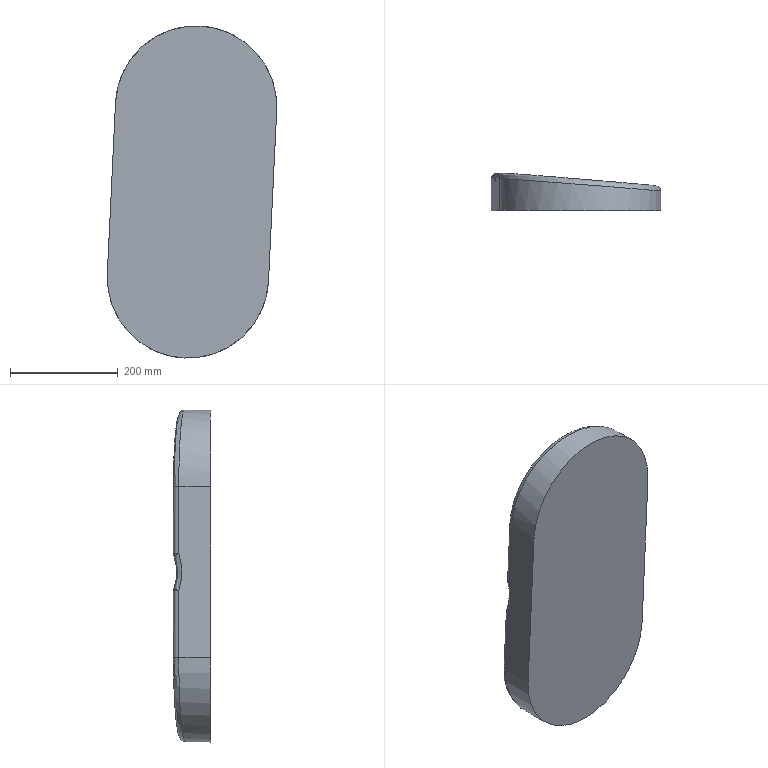Component | SolidWorks | 04-03BottomHousing-1 | 1 solid | 22 faces | box 315.25 x 69.13 x 617.63 mm | volume 9437459 mm3 | cylinder 9 | plane 5 | sphere 4 | spline 4 | commonest cylinder face diameters 20 x6 300 x2 180 x1
STEP:
#1=COLOUR_RGB('',0.7922,0.8196,0.9333);
#2=FILL_AREA_STYLE_COLOUR('',#1);
#3=FILL_AREA_STYLE('',(#2));
#4=SURFACE_STYLE_FILL_AREA(#3);
#5=SURFACE_SIDE_STYLE('',(#4));
#6=SURFACE_STYLE_USAGE(.BOTH.,#5);
#7=PRESENTATION_STYLE_ASSIGNMENT((#6));
#8=CARTESIAN_POINT('',(2.905,4.413,6.332));
#9=VERTEX_POINT('',#8);
#10=CARTESIAN_POINT('',(13.916,3.495,5.804));
#11=VERTEX_POINT('',#10);
#12=CARTESIAN_POINT('',(2.905,4.413,6.332));
#13=CARTESIAN_POINT('',(3.434,4.413,17.343));
#14=CARTESIAN_POINT('',(14.444,3.495,16.815));
#15=CARTESIAN_POINT('',(13.916,3.495,5.804));
#16=(BOUNDED_CURVE()B_SPLINE_CURVE(3,(#12,#13,#14,#15),.UNSPECIFIED.,.F.,.F.)B_SPLINE_CURVE_WITH_KNOTS((4,4),(3.142,6.283),.UNSPECIFIED.)CURVE()GEOMETRIC_REPRESENTATION_ITEM()RATIONAL_B_SPLINE_CURVE((1.,0.3333,0.3333,1.))REPRESENTATION_ITEM(''));
#17=EDGE_CURVE('',#9,#11,#16,.T.);
#18=ORIENTED_EDGE('',*,*,#17,.T.);
#19=CARTESIAN_POINT('',(13.68,3.495,0.8927));
#20=VERTEX_POINT('',#19);
#21=CARTESIAN_POINT('',(14.199,3.495,11.702));
#22=DIRECTION('',(-0.04795,-0.,-0.9988));
#23=VECTOR('',#22,39.37);
#24=LINE('',#21,#23);
#25=EDGE_CURVE('',#11,#20,#24,.T.);
#26=ORIENTED_EDGE('',*,*,#25,.T.);
#27=CARTESIAN_POINT('',(2.669,4.413,1.421));
#28=VERTEX_POINT('',#27);
#29=CARTESIAN_POINT('',(2.243,4.449,1.442));
#30=DIRECTION('',(-0.9954,0.08305,0.04778));
#31=VECTOR('',#30,39.37);
#32=LINE('',#29,#31);
#33=EDGE_CURVE('',#20,#28,#32,.T.);
#34=ORIENTED_EDGE('',*,*,#33,.T.);
#35=CARTESIAN_POINT('',(3.188,4.413,12.231));
#36=DIRECTION('',(0.04795,0.,0.9988));
#37=VECTOR('',#36,39.37);
#38=LINE('',#35,#37);
#39=EDGE_CURVE('',#28,#9,#38,.T.);
#40=ORIENTED_EDGE('',*,*,#39,.T.);
#41=EDGE_LOOP('',(#18,#26,#34,#40));
#42=FACE_OUTER_BOUND('',#41,.T.);
#43=CARTESIAN_POINT('',(2.762,4.449,12.251));
#44=DIRECTION('',(-0.08295,-0.9965,0.003982));
#45=DIRECTION('',(-0.9954,0.08305,0.04778));
#46=AXIS2_PLACEMENT_3D('',#43,#44,#45);
#47=PLANE('',#46);
#48=ADVANCED_FACE('',(#42),#47,.F.);
#49=CARTESIAN_POINT('',(13.316,3.495,-6.702));
#50=VERTEX_POINT('',#49);
#51=CARTESIAN_POINT('',(2.305,4.413,-6.173));
#52=VERTEX_POINT('',#51);
#53=CARTESIAN_POINT('',(13.316,3.495,-6.702));
#54=CARTESIAN_POINT('',(12.787,3.495,-17.713));
#55=CARTESIAN_POINT('',(1.776,4.413,-17.184));
#56=CARTESIAN_POINT('',(2.305,4.413,-6.173));
#57=(BOUNDED_CURVE()B_SPLINE_CURVE(3,(#53,#54,#55,#56),.UNSPECIFIED.,.F.,.F.)B_SPLINE_CURVE_WITH_KNOTS((4,4),(0.,3.142),.UNSPECIFIED.)CURVE()GEOMETRIC_REPRESENTATION_ITEM()RATIONAL_B_SPLINE_CURVE((1.,0.3333,0.3333,1.))REPRESENTATION_ITEM(''));
#58=EDGE_CURVE('',#50,#52,#57,.T.);
#59=ORIENTED_EDGE('',*,*,#58,.T.);
#60=CARTESIAN_POINT('',(2.54,4.413,-1.262));
#61=VERTEX_POINT('',#60);
#62=CARTESIAN_POINT('',(3.188,4.413,12.231));
#63=DIRECTION('',(0.04795,0.,0.9988));
#64=VECTOR('',#63,39.37);
#65=LINE('',#62,#64);
#66=EDGE_CURVE('',#52,#61,#65,.T.);
#67=ORIENTED_EDGE('',*,*,#66,.T.);
#68=CARTESIAN_POINT('',(13.551,3.495,-1.791));
#69=VERTEX_POINT('',#68);
#70=CARTESIAN_POINT('',(13.912,3.465,-1.808));
#71=DIRECTION('',(0.9954,-0.08305,-0.04778));
#72=VECTOR('',#71,39.37);
#73=LINE('',#70,#72);
#74=EDGE_CURVE('',#61,#69,#73,.T.);
#75=ORIENTED_EDGE('',*,*,#74,.T.);
#76=CARTESIAN_POINT('',(14.199,3.495,11.702));
#77=DIRECTION('',(-0.04795,-0.,-0.9988));
#78=VECTOR('',#77,39.37);
#79=LINE('',#76,#78);
#80=EDGE_CURVE('',#69,#50,#79,.T.);
#81=ORIENTED_EDGE('',*,*,#80,.T.);
#82=EDGE_LOOP('',(#59,#67,#75,#81));
#83=FACE_OUTER_BOUND('',#82,.T.);
#84=CARTESIAN_POINT('',(2.762,4.449,12.251));
#85=DIRECTION('',(-0.08295,-0.9965,0.003982));
#86=DIRECTION('',(-0.9954,0.08305,0.04778));
#87=AXIS2_PLACEMENT_3D('',#84,#85,#86);
#88=PLANE('',#87);
#89=ADVANCED_FACE('',(#83),#88,.F.);
#90=CARTESIAN_POINT('',(1.879,4.021,-6.153));
#91=VERTEX_POINT('',#90);
#92=CARTESIAN_POINT('',(1.879,1.693,-6.153));
#93=VERTEX_POINT('',#92);
#94=CARTESIAN_POINT('',(1.879,5.236,-6.153));
#95=DIRECTION('',(0.,-1.,0.));
#96=VECTOR('',#95,39.37);
#97=LINE('',#94,#96);
#98=EDGE_CURVE('',#91,#93,#97,.T.);
#99=ORIENTED_EDGE('',*,*,#98,.F.);
#100=CARTESIAN_POINT('',(13.676,3.102,-6.719));
#101=VERTEX_POINT('',#100);
#102=CARTESIAN_POINT('',(1.879,4.021,-6.153));
#103=CARTESIAN_POINT('',(1.312,4.021,-17.95));
#104=CARTESIAN_POINT('',(13.11,3.102,-18.516));
#105=CARTESIAN_POINT('',(13.676,3.102,-6.719));
#106=(BOUNDED_CURVE()B_SPLINE_CURVE(3,(#102,#103,#104,#105),.UNSPECIFIED.,.F.,.T.)B_SPLINE_CURVE_WITH_KNOTS((4,4),(3.142,6.283),.UNSPECIFIED.)CURVE()GEOMETRIC_REPRESENTATION_ITEM()RATIONAL_B_SPLINE_CURVE((1.,0.3333,0.3333,1.))REPRESENTATION_ITEM(''));
#107=EDGE_CURVE('',#91,#101,#106,.T.);
#108=ORIENTED_EDGE('',*,*,#107,.T.);
#109=CARTESIAN_POINT('',(13.676,1.693,-6.719));
#110=VERTEX_POINT('',#109);
#111=CARTESIAN_POINT('',(13.676,5.236,-6.719));
#112=DIRECTION('',(0.,-1.,0.));
#113=VECTOR('',#112,39.37);
#114=LINE('',#111,#113);
#115=EDGE_CURVE('',#101,#110,#114,.T.);
#116=ORIENTED_EDGE('',*,*,#115,.T.);
#117=CARTESIAN_POINT('',(7.777,1.693,-6.436));
#118=DIRECTION('',(-0.,1.,-0.));
#119=DIRECTION('',(0.9988,0.,-0.04795));
#120=AXIS2_PLACEMENT_3D('',#117,#118,#119);
#121=CIRCLE('',#120,5.906);
#122=EDGE_CURVE('',#110,#93,#121,.T.);
#123=ORIENTED_EDGE('',*,*,#122,.T.);
#124=EDGE_LOOP('',(#99,#108,#116,#123));
#125=FACE_OUTER_BOUND('',#124,.T.);
#126=CARTESIAN_POINT('',(7.777,5.236,-6.436));
#127=DIRECTION('',(0.,-1.,0.));
#128=DIRECTION('',(-0.9988,-0.,0.04795));
#129=AXIS2_PLACEMENT_3D('',#126,#127,#128);
#130=CYLINDRICAL_SURFACE('',#129,5.906);
#131=ADVANCED_FACE('',(#125),#130,.T.);
#132=CARTESIAN_POINT('',(2.479,4.021,6.353));
#133=VERTEX_POINT('',#132);
#134=CARTESIAN_POINT('',(2.479,1.693,6.353));
#135=VERTEX_POINT('',#134);
#136=CARTESIAN_POINT('',(2.479,5.236,6.353));
#137=DIRECTION('',(0.,-1.,0.));
#138=VECTOR('',#137,39.37);
#139=LINE('',#136,#138);
#140=EDGE_CURVE('',#133,#135,#139,.T.);
#141=ORIENTED_EDGE('',*,*,#140,.F.);
#142=CARTESIAN_POINT('',(2.243,4.021,1.442));
#143=VERTEX_POINT('',#142);
#144=CARTESIAN_POINT('',(1.879,4.021,-6.153));
#145=DIRECTION('',(-0.04795,-0.,-0.9988));
#146=VECTOR('',#145,39.37);
#147=LINE('',#144,#146);
#148=EDGE_CURVE('',#133,#143,#147,.T.);
#149=ORIENTED_EDGE('',*,*,#148,.T.);
#150=CARTESIAN_POINT('',(2.114,4.021,-1.242));
#151=VERTEX_POINT('',#150);
#152=CARTESIAN_POINT('',(2.243,4.021,1.442));
#153=CARTESIAN_POINT('',(2.201,3.702,0.5659));
#154=CARTESIAN_POINT('',(2.157,3.702,-0.3658));
#155=CARTESIAN_POINT('',(2.114,4.021,-1.242));
#156=(BOUNDED_CURVE()B_SPLINE_CURVE(3,(#152,#153,#154,#155),.UNSPECIFIED.,.F.,.F.)B_SPLINE_CURVE_WITH_KNOTS((4,4),(2.793,3.49),.UNSPECIFIED.)CURVE()GEOMETRIC_REPRESENTATION_ITEM()RATIONAL_B_SPLINE_CURVE((1.,0.96,0.96,1.))REPRESENTATION_ITEM(''));
#157=EDGE_CURVE('',#143,#151,#156,.T.);
#158=ORIENTED_EDGE('',*,*,#157,.T.);
#159=CARTESIAN_POINT('',(1.879,4.021,-6.153));
#160=DIRECTION('',(-0.04795,-0.,-0.9988));
#161=VECTOR('',#160,39.37);
#162=LINE('',#159,#161);
#163=EDGE_CURVE('',#151,#91,#162,.T.);
#164=ORIENTED_EDGE('',*,*,#163,.T.);
#165=ORIENTED_EDGE('',*,*,#98,.T.);
#166=CARTESIAN_POINT('',(1.879,1.693,-6.153));
#167=DIRECTION('',(0.04795,0.,0.9988));
#168=VECTOR('',#167,39.37);
#169=LINE('',#166,#168);
#170=EDGE_CURVE('',#93,#135,#169,.T.);
#171=ORIENTED_EDGE('',*,*,#170,.T.);
#172=EDGE_LOOP('',(#141,#149,#158,#164,#165,#171));
#173=FACE_OUTER_BOUND('',#172,.T.);
#174=CARTESIAN_POINT('',(1.879,5.236,-6.153));
#175=DIRECTION('',(0.9988,0.,-0.04795));
#176=DIRECTION('',(-0.04795,-0.,-0.9988));
#177=AXIS2_PLACEMENT_3D('',#174,#175,#176);
#178=PLANE('',#177);
#179=ADVANCED_FACE('',(#173),#178,.F.);
#180=CARTESIAN_POINT('',(14.276,3.102,5.786));
#181=VERTEX_POINT('',#180);
#182=CARTESIAN_POINT('',(14.276,1.693,5.786));
#183=VERTEX_POINT('',#182);
#184=CARTESIAN_POINT('',(14.276,5.236,5.786));
#185=DIRECTION('',(0.,-1.,0.));
#186=VECTOR('',#185,39.37);
#187=LINE('',#184,#186);
#188=EDGE_CURVE('',#181,#183,#187,.T.);
#189=ORIENTED_EDGE('',*,*,#188,.F.);
#190=CARTESIAN_POINT('',(14.276,3.102,5.786));
#191=CARTESIAN_POINT('',(14.843,3.102,17.584));
#192=CARTESIAN_POINT('',(3.045,4.021,18.15));
#193=CARTESIAN_POINT('',(2.479,4.021,6.353));
#194=(BOUNDED_CURVE()B_SPLINE_CURVE(3,(#190,#191,#192,#193),.UNSPECIFIED.,.F.,.F.)B_SPLINE_CURVE_WITH_KNOTS((4,4),(0.,3.142),.UNSPECIFIED.)CURVE()GEOMETRIC_REPRESENTATION_ITEM()RATIONAL_B_SPLINE_CURVE((1.,0.3333,0.3333,1.))REPRESENTATION_ITEM(''));
#195=EDGE_CURVE('',#181,#133,#194,.T.);
#196=ORIENTED_EDGE('',*,*,#195,.T.);
#197=ORIENTED_EDGE('',*,*,#140,.T.);
#198=CARTESIAN_POINT('',(8.378,1.693,6.07));
#199=DIRECTION('',(-0.,1.,-0.));
#200=DIRECTION('',(0.9988,0.,-0.04795));
#201=AXIS2_PLACEMENT_3D('',#198,#199,#200);
#202=CIRCLE('',#201,5.906);
#203=EDGE_CURVE('',#135,#183,#202,.T.);
#204=ORIENTED_EDGE('',*,*,#203,.T.);
#205=EDGE_LOOP('',(#189,#196,#197,#204));
#206=FACE_OUTER_BOUND('',#205,.T.);
#207=CARTESIAN_POINT('',(8.378,5.236,6.07));
#208=DIRECTION('',(0.,-1.,0.));
#209=DIRECTION('',(-0.9988,-0.,0.04795));
#210=AXIS2_PLACEMENT_3D('',#207,#208,#209);
#211=CYLINDRICAL_SURFACE('',#210,5.906);
#212=ADVANCED_FACE('',(#206),#211,.T.);
#213=CARTESIAN_POINT('',(13.912,3.102,-1.808));
#214=VERTEX_POINT('',#213);
#215=CARTESIAN_POINT('',(14.041,3.102,0.8754));
#216=VERTEX_POINT('',#215);
#217=CARTESIAN_POINT('',(13.912,3.102,-1.808));
#218=CARTESIAN_POINT('',(13.954,2.783,-0.9321));
#219=CARTESIAN_POINT('',(13.999,2.783,-0.0004051));
#220=CARTESIAN_POINT('',(14.041,3.102,0.8754));
#221=(BOUNDED_CURVE()B_SPLINE_CURVE(3,(#217,#218,#219,#220),.UNSPECIFIED.,.F.,.F.)B_SPLINE_CURVE_WITH_KNOTS((4,4),(2.793,3.49),.UNSPECIFIED.)CURVE()GEOMETRIC_REPRESENTATION_ITEM()RATIONAL_B_SPLINE_CURVE((1.,0.96,0.96,1.))REPRESENTATION_ITEM(''));
#222=EDGE_CURVE('',#214,#216,#221,.T.);
#223=ORIENTED_EDGE('',*,*,#222,.T.);
#224=CARTESIAN_POINT('',(13.676,3.102,-6.719));
#225=DIRECTION('',(0.04795,0.,0.9988));
#226=VECTOR('',#225,39.37);
#227=LINE('',#224,#226);
#228=EDGE_CURVE('',#216,#181,#227,.T.);
#229=ORIENTED_EDGE('',*,*,#228,.T.);
#230=ORIENTED_EDGE('',*,*,#188,.T.);
#231=CARTESIAN_POINT('',(13.676,1.693,-6.719));
#232=DIRECTION('',(-0.04795,-0.,-0.9988));
#233=VECTOR('',#232,39.37);
#234=LINE('',#231,#233);
#235=EDGE_CURVE('',#183,#110,#234,.T.);
#236=ORIENTED_EDGE('',*,*,#235,.T.);
#237=ORIENTED_EDGE('',*,*,#115,.F.);
#238=CARTESIAN_POINT('',(13.676,3.102,-6.719));
#239=DIRECTION('',(0.04795,0.,0.9988));
#240=VECTOR('',#239,39.37);
#241=LINE('',#238,#240);
#242=EDGE_CURVE('',#101,#214,#241,.T.);
#243=ORIENTED_EDGE('',*,*,#242,.T.);
#244=EDGE_LOOP('',(#223,#229,#230,#236,#237,#243));
#245=FACE_OUTER_BOUND('',#244,.T.);
#246=CARTESIAN_POINT('',(13.676,5.236,-6.719));
#247=DIRECTION('',(-0.9988,-0.,0.04795));
#248=DIRECTION('',(0.04795,0.,0.9988));
#249=AXIS2_PLACEMENT_3D('',#246,#247,#248);
#250=PLANE('',#249);
#251=ADVANCED_FACE('',(#245),#250,.F.);
#252=ORIENTED_EDGE('',*,*,#122,.F.);
#253=ORIENTED_EDGE('',*,*,#235,.F.);
#254=ORIENTED_EDGE('',*,*,#203,.F.);
#255=ORIENTED_EDGE('',*,*,#170,.F.);
#256=EDGE_LOOP('',(#252,#253,#254,#255));
#257=FACE_OUTER_BOUND('',#256,.T.);
#258=CARTESIAN_POINT('',(7.777,1.693,-6.436));
#259=DIRECTION('',(-0.,1.,-0.));
#260=DIRECTION('',(0.9988,0.,-0.04795));
#261=AXIS2_PLACEMENT_3D('',#258,#259,#260);
#262=PLANE('',#261);
#263=ADVANCED_FACE('',(#257),#262,.F.);
#264=CARTESIAN_POINT('',(2.545,4.39,-1.128));
#265=VERTEX_POINT('',#264);
#266=CARTESIAN_POINT('',(2.661,4.39,1.287));
#267=VERTEX_POINT('',#266);
#268=CARTESIAN_POINT('',(2.545,4.39,-1.128));
#269=CARTESIAN_POINT('',(2.585,4.102,-0.3397));
#270=CARTESIAN_POINT('',(2.626,4.102,0.4989));
#271=CARTESIAN_POINT('',(2.661,4.39,1.287));
#272=(BOUNDED_CURVE()B_SPLINE_CURVE(3,(#268,#269,#270,#271),.UNSPECIFIED.,.F.,.T.)B_SPLINE_CURVE_WITH_KNOTS((4,4),(2.793,3.49),.UNSPECIFIED.)CURVE()GEOMETRIC_REPRESENTATION_ITEM()RATIONAL_B_SPLINE_CURVE((1.,0.96,0.96,1.))REPRESENTATION_ITEM(''));
#273=EDGE_CURVE('',#265,#267,#272,.T.);
#274=ORIENTED_EDGE('',*,*,#273,.T.);
#275=CARTESIAN_POINT('',(13.672,3.471,0.7586));
#276=VERTEX_POINT('',#275);
#277=CARTESIAN_POINT('',(1.297,4.504,1.353));
#278=DIRECTION('',(0.9954,-0.08305,-0.04778));
#279=VECTOR('',#278,39.37);
#280=LINE('',#277,#279);
#281=EDGE_CURVE('',#267,#276,#280,.T.);
#282=ORIENTED_EDGE('',*,*,#281,.T.);
#283=CARTESIAN_POINT('',(13.556,3.471,-1.656));
#284=VERTEX_POINT('',#283);
#285=CARTESIAN_POINT('',(13.672,3.471,0.7586));
#286=CARTESIAN_POINT('',(13.637,3.183,-0.02971));
#287=CARTESIAN_POINT('',(13.596,3.183,-0.8683));
#288=CARTESIAN_POINT('',(13.556,3.471,-1.656));
#289=(BOUNDED_CURVE()B_SPLINE_CURVE(3,(#285,#286,#287,#288),.UNSPECIFIED.,.F.,.F.)B_SPLINE_CURVE_WITH_KNOTS((4,4),(2.793,3.49),.UNSPECIFIED.)CURVE()GEOMETRIC_REPRESENTATION_ITEM()RATIONAL_B_SPLINE_CURVE((1.,0.96,0.96,1.))REPRESENTATION_ITEM(''));
#290=EDGE_CURVE('',#276,#284,#289,.T.);
#291=ORIENTED_EDGE('',*,*,#290,.T.);
#292=CARTESIAN_POINT('',(1.181,4.504,-1.062));
#293=DIRECTION('',(-0.9954,0.08305,0.04778));
#294=VECTOR('',#293,39.37);
#295=LINE('',#292,#294);
#296=EDGE_CURVE('',#284,#265,#295,.T.);
#297=ORIENTED_EDGE('',*,*,#296,.T.);
#298=EDGE_LOOP('',(#274,#282,#291,#297));
#299=FACE_OUTER_BOUND('',#298,.T.);
#300=CARTESIAN_POINT('',(1.515,7.823,0.1319));
#301=DIRECTION('',(-0.9954,0.08305,0.04778));
#302=DIRECTION('',(0.08295,0.9965,-0.003982));
#303=AXIS2_PLACEMENT_3D('',#300,#301,#302);
#304=CYLINDRICAL_SURFACE('',#303,3.543);
#305=ADVANCED_FACE('',(#299),#304,.F.);
#306=CARTESIAN_POINT('',(2.508,4.021,-1.26));
#307=DIRECTION('',(0.04795,-0.,0.9988));
#308=DIRECTION('',(0.9988,0.,-0.04795));
#309=AXIS2_PLACEMENT_3D('',#306,#307,#308);
#310=CIRCLE('',#309,0.3937);
#311=EDGE_CURVE('',#61,#151,#310,.T.);
#312=ORIENTED_EDGE('',*,*,#311,.F.);
#313=ORIENTED_EDGE('',*,*,#66,.F.);
#314=CARTESIAN_POINT('',(2.272,4.021,-6.171));
#315=DIRECTION('',(-0.04795,-0.,-0.9988));
#316=DIRECTION('',(-0.9988,0.,0.04795));
#317=AXIS2_PLACEMENT_3D('',#314,#315,#316);
#318=CIRCLE('',#317,0.3937);
#319=EDGE_CURVE('',#91,#52,#318,.T.);
#320=ORIENTED_EDGE('',*,*,#319,.F.);
#321=ORIENTED_EDGE('',*,*,#163,.F.);
#322=EDGE_LOOP('',(#312,#313,#320,#321));
#323=FACE_OUTER_BOUND('',#322,.T.);
#324=CARTESIAN_POINT('',(2.272,4.021,-6.171));
#325=DIRECTION('',(-0.04795,-0.,-0.9988));
#326=DIRECTION('',(-0.9988,0.,0.04795));
#327=AXIS2_PLACEMENT_3D('',#324,#325,#326);
#328=CYLINDRICAL_SURFACE('',#327,0.3937);
#329=ADVANCED_FACE('',(#323),#328,.T.);
#330=CARTESIAN_POINT('',(2.508,4.021,-1.26));
#331=DIRECTION('',(0.9954,-0.08305,-0.04778));
#332=DIRECTION('',(0.08295,0.9965,-0.003982));
#333=AXIS2_PLACEMENT_3D('',#330,#331,#332);
#334=CIRCLE('',#333,0.3937);
#335=EDGE_CURVE('',#61,#265,#334,.T.);
#336=ORIENTED_EDGE('',*,*,#335,.F.);
#337=ORIENTED_EDGE('',*,*,#311,.T.);
#338=CARTESIAN_POINT('',(2.508,4.021,-1.26));
#339=DIRECTION('',(0.04505,-0.3422,0.9385));
#340=DIRECTION('',(0.01641,0.9396,0.3418));
#341=AXIS2_PLACEMENT_3D('',#338,#339,#340);
#342=CIRCLE('',#341,0.3937);
#343=EDGE_CURVE('',#265,#151,#342,.T.);
#344=ORIENTED_EDGE('',*,*,#343,.F.);
#345=EDGE_LOOP('',(#336,#337,#344));
#346=FACE_OUTER_BOUND('',#345,.T.);
#347=CARTESIAN_POINT('',(2.508,4.021,-1.26));
#348=DIRECTION('',(-0.,1.,0.));
#349=DIRECTION('',(-0.04795,0.,-0.9988));
#350=AXIS2_PLACEMENT_3D('',#347,#348,#349);
#351=SPHERICAL_SURFACE('',#350,0.3937);
#352=ADVANCED_FACE('',(#346),#351,.T.);
#353=ORIENTED_EDGE('',*,*,#319,.T.);
#354=ORIENTED_EDGE('',*,*,#58,.F.);
#355=CARTESIAN_POINT('',(13.283,3.102,-6.7));
#356=DIRECTION('',(0.04795,0.,0.9988));
#357=DIRECTION('',(0.9988,0.,-0.04795));
#358=AXIS2_PLACEMENT_3D('',#355,#356,#357);
#359=CIRCLE('',#358,0.3937);
#360=EDGE_CURVE('',#101,#50,#359,.T.);
#361=ORIENTED_EDGE('',*,*,#360,.F.);
#362=ORIENTED_EDGE('',*,*,#107,.F.);
#363=EDGE_LOOP('',(#353,#354,#361,#362));
#364=FACE_OUTER_BOUND('',#363,.T.);
#365=CARTESIAN_POINT('',(2.305,4.413,-6.173));
#366=CARTESIAN_POINT('',(1.879,4.449,-6.153));
#367=CARTESIAN_POINT('',(1.879,4.021,-6.153));
#368=CARTESIAN_POINT('',(2.287,4.413,-6.533));
#369=CARTESIAN_POINT('',(1.86,4.449,-6.541));
#370=CARTESIAN_POINT('',(1.86,4.021,-6.539));
#371=CARTESIAN_POINT('',(2.306,4.41,-6.895));
#372=CARTESIAN_POINT('',(1.88,4.446,-6.931));
#373=CARTESIAN_POINT('',(1.88,4.018,-6.927));
#374=CARTESIAN_POINT('',(2.412,4.399,-7.609));
#375=CARTESIAN_POINT('',(1.996,4.433,-7.7));
#376=CARTESIAN_POINT('',(1.994,4.006,-7.691));
#377=CARTESIAN_POINT('',(2.501,4.39,-7.96));
#378=CARTESIAN_POINT('',(2.092,4.423,-8.078));
#379=CARTESIAN_POINT('',(2.089,3.997,-8.068));
#380=CARTESIAN_POINT('',(2.744,4.367,-8.64));
#381=CARTESIAN_POINT('',(2.356,4.398,-8.809));
#382=CARTESIAN_POINT('',(2.35,3.974,-8.795));
#383=CARTESIAN_POINT('',(2.9,4.353,-8.967));
#384=CARTESIAN_POINT('',(2.524,4.383,-9.161));
#385=CARTESIAN_POINT('',(2.516,3.96,-9.146));
#386=CARTESIAN_POINT('',(3.271,4.319,-9.585));
#387=CARTESIAN_POINT('',(2.926,4.347,-9.826));
#388=CARTESIAN_POINT('',(2.915,3.927,-9.809));
#389=CARTESIAN_POINT('',(3.488,4.3,-9.876));
#390=CARTESIAN_POINT('',(3.16,4.326,-10.138));
#391=CARTESIAN_POINT('',(3.146,3.908,-10.12));
#392=CARTESIAN_POINT('',(3.973,4.257,-10.41));
#393=CARTESIAN_POINT('',(3.684,4.28,-10.71));
#394=CARTESIAN_POINT('',(3.666,3.865,-10.693));
#395=CARTESIAN_POINT('',(4.242,4.234,-10.654));
#396=CARTESIAN_POINT('',(3.974,4.255,-10.97));
#397=CARTESIAN_POINT('',(3.954,3.842,-10.953));
#398=CARTESIAN_POINT('',(4.822,4.184,-11.083));
#399=CARTESIAN_POINT('',(4.6,4.201,-11.428));
#400=CARTESIAN_POINT('',(4.576,3.792,-11.413));
#401=CARTESIAN_POINT('',(5.133,4.158,-11.269));
#402=CARTESIAN_POINT('',(4.935,4.173,-11.627));
#403=CARTESIAN_POINT('',(4.909,3.765,-11.612));
#404=CARTESIAN_POINT('',(5.785,4.102,-11.576));
#405=CARTESIAN_POINT('',(5.637,4.113,-11.953));
#406=CARTESIAN_POINT('',(5.608,3.71,-11.942));
#407=CARTESIAN_POINT('',(6.127,4.073,-11.698));
#408=CARTESIAN_POINT('',(6.004,4.082,-12.082));
#409=CARTESIAN_POINT('',(5.974,3.681,-12.072));
#410=CARTESIAN_POINT('',(6.827,4.014,-11.873));
#411=CARTESIAN_POINT('',(6.755,4.018,-12.265));
#412=CARTESIAN_POINT('',(6.724,3.622,-12.259));
#413=CARTESIAN_POINT('',(7.185,3.984,-11.925));
#414=CARTESIAN_POINT('',(7.14,3.986,-12.32));
#415=CARTESIAN_POINT('',(7.108,3.592,-12.316));
#416=CARTESIAN_POINT('',(7.906,3.924,-11.96));
#417=CARTESIAN_POINT('',(7.912,3.922,-12.352));
#418=CARTESIAN_POINT('',(7.88,3.532,-12.353));
#419=CARTESIAN_POINT('',(8.268,3.894,-11.942));
#420=CARTESIAN_POINT('',(8.299,3.89,-12.331));
#421=CARTESIAN_POINT('',(8.268,3.502,-12.333));
#422=CARTESIAN_POINT('',(8.982,3.835,-11.835));
#423=CARTESIAN_POINT('',(9.062,3.827,-12.213));
#424=CARTESIAN_POINT('',(9.033,3.443,-12.219));
#425=CARTESIAN_POINT('',(9.333,3.806,-11.747));
#426=CARTESIAN_POINT('',(9.438,3.796,-12.116));
#427=CARTESIAN_POINT('',(9.409,3.414,-12.124));
#428=CARTESIAN_POINT('',(10.012,3.75,-11.503));
#429=CARTESIAN_POINT('',(10.162,3.737,-11.852));
#430=CARTESIAN_POINT('',(10.137,3.358,-11.863));
#431=CARTESIAN_POINT('',(10.34,3.724,-11.348));
#432=CARTESIAN_POINT('',(10.511,3.708,-11.685));
#433=CARTESIAN_POINT('',(10.488,3.331,-11.697));
#434=CARTESIAN_POINT('',(10.958,3.674,-10.976));
#435=CARTESIAN_POINT('',(11.17,3.655,-11.285));
#436=CARTESIAN_POINT('',(11.15,3.281,-11.299));
#437=CARTESIAN_POINT('',(11.249,3.65,-10.76));
#438=CARTESIAN_POINT('',(11.48,3.63,-11.053));
#439=CARTESIAN_POINT('',(11.462,3.258,-11.067));
#440=CARTESIAN_POINT('',(11.783,3.608,-10.275));
#441=CARTESIAN_POINT('',(12.048,3.585,-10.533));
#442=CARTESIAN_POINT('',(12.034,3.216,-10.547));
#443=CARTESIAN_POINT('',(12.026,3.589,-10.006));
#444=CARTESIAN_POINT('',(12.307,3.564,-10.245));
#445=CARTESIAN_POINT('',(12.295,3.196,-10.259));
#446=CARTESIAN_POINT('',(12.455,3.555,-9.426));
#447=CARTESIAN_POINT('',(12.763,3.529,-9.625));
#448=CARTESIAN_POINT('',(12.755,3.163,-9.638));
#449=CARTESIAN_POINT('',(12.641,3.541,-9.115));
#450=CARTESIAN_POINT('',(12.96,3.514,-9.293));
#451=CARTESIAN_POINT('',(12.954,3.149,-9.304));
#452=CARTESIAN_POINT('',(12.949,3.518,-8.462));
#453=CARTESIAN_POINT('',(13.287,3.489,-8.596));
#454=CARTESIAN_POINT('',(13.284,3.126,-8.605));
#455=CARTESIAN_POINT('',(13.071,3.509,-8.121));
#456=CARTESIAN_POINT('',(13.416,3.48,-8.232));
#457=CARTESIAN_POINT('',(13.414,3.117,-8.239));
#458=CARTESIAN_POINT('',(13.246,3.498,-7.421));
#459=CARTESIAN_POINT('',(13.602,3.468,-7.485));
#460=CARTESIAN_POINT('',(13.601,3.105,-7.489));
#461=CARTESIAN_POINT('',(13.298,3.495,-7.062));
#462=CARTESIAN_POINT('',(13.658,3.465,-7.103));
#463=CARTESIAN_POINT('',(13.658,3.102,-7.105));
#464=CARTESIAN_POINT('',(13.316,3.495,-6.702));
#465=CARTESIAN_POINT('',(13.676,3.465,-6.719));
#466=CARTESIAN_POINT('',(13.676,3.102,-6.719));
#467=(BOUNDED_SURFACE()B_SPLINE_SURFACE(3,2,((#365,#366,#367),(#368,#369,#370),(#371,#372,#373),(#374,#375,#376),(#377,#378,#379),(#380,#381,#382),(#383,#384,#385),(#386,#387,#388),(#389,#390,#391),(#392,#393,#394),(#395,#396,#397),(#398,#399,#400),(#401,#402,#403),(#404,#405,#406),(#407,#408,#409),(#410,#411,#412),(#413,#414,#415),(#416,#417,#418),(#419,#420,#421),(#422,#423,#424),(#425,#426,#427),(#428,#429,#430),(#431,#432,#433),(#434,#435,#436),(#437,#438,#439),(#440,#441,#442),(#443,#444,#445),(#446,#447,#448),(#449,#450,#451),(#452,#453,#454),(#455,#456,#457),(#458,#459,#460),(#461,#462,#463),(#464,#465,#466)),.UNSPECIFIED.,.F.,.F.,.T.)B_SPLINE_SURFACE_WITH_KNOTS((4,2,2,2,2,2,2,2,2,2,2,2,2,2,2,2,4),(3,3),(3.142,3.338,3.534,3.731,3.927,4.123,4.32,4.516,4.712,4.909,5.105,5.301,5.498,5.694,5.89,6.087,6.283),(0.,1.),.UNSPECIFIED.)GEOMETRIC_REPRESENTATION_ITEM()RATIONAL_B_SPLINE_SURFACE(((1.,0.6771,1.),(1.,0.6771,1.),(1.,0.6773,1.),(1.,0.6781,1.),(1.,0.6787,1.),(1.,0.6802,1.),(1.,0.6812,1.),(1.,0.6834,1.),(1.,0.6846,1.),(1.,0.6874,1.),(1.,0.689,1.),(1.,0.6922,1.),(1.,0.694,1.),(1.,0.6976,1.),(1.,0.6995,1.),(1.,0.7033,1.),(1.,0.7052,1.),(1.,0.709,1.),(1.,0.7109,1.),(1.,0.7147,1.),(1.,0.7165,1.),(1.,0.72,1.),(1.,0.7217,1.),(1.,0.7248,1.),(1.,0.7263,1.),(1.,0.7289,1.),(1.,0.7301,1.),(1.,0.7321,1.),(1.,0.733,1.),(1.,0.7344,1.),(1.,0.735,1.),(1.,0.7357,1.),(1.,0.7359,1.),(1.,0.7359,1.)))REPRESENTATION_ITEM('')SURFACE());
#468=ADVANCED_FACE('',(#364),#467,.T.);
#469=ORIENTED_EDGE('',*,*,#343,.T.);
#470=ORIENTED_EDGE('',*,*,#157,.F.);
#471=CARTESIAN_POINT('',(2.637,4.021,1.423));
#472=DIRECTION('',(0.04505,0.3422,0.9385));
#473=DIRECTION('',(0.01641,-0.9396,0.3418));
#474=AXIS2_PLACEMENT_3D('',#471,#472,#473);
#475=CIRCLE('',#474,0.3937);
#476=EDGE_CURVE('',#267,#143,#475,.T.);
#477=ORIENTED_EDGE('',*,*,#476,.F.);
#478=ORIENTED_EDGE('',*,*,#273,.F.);
#479=EDGE_LOOP('',(#469,#470,#477,#478));
#480=FACE_OUTER_BOUND('',#479,.T.);
#481=CARTESIAN_POINT('',(2.661,4.39,1.287));
#482=CARTESIAN_POINT('',(2.236,4.421,1.296));
#483=CARTESIAN_POINT('',(2.243,4.021,1.442));
#484=CARTESIAN_POINT('',(2.652,4.319,1.094));
#485=CARTESIAN_POINT('',(2.227,4.352,1.105));
#486=CARTESIAN_POINT('',(2.233,3.943,1.227));
#487=CARTESIAN_POINT('',(2.643,4.266,0.895));
#488=CARTESIAN_POINT('',(2.218,4.299,0.9073));
#489=CARTESIAN_POINT('',(2.222,3.883,1.006));
#490=CARTESIAN_POINT('',(2.624,4.194,0.4904));
#491=CARTESIAN_POINT('',(2.198,4.229,0.5066));
#492=CARTESIAN_POINT('',(2.201,3.804,0.5565));
#493=CARTESIAN_POINT('',(2.615,4.176,0.285));
#494=CARTESIAN_POINT('',(2.189,4.212,0.3034));
#495=CARTESIAN_POINT('',(2.19,3.784,0.3283));
#496=CARTESIAN_POINT('',(2.595,4.176,-0.1257));
#497=CARTESIAN_POINT('',(2.169,4.212,-0.1032));
#498=CARTESIAN_POINT('',(2.168,3.784,-0.1281));
#499=CARTESIAN_POINT('',(2.585,4.194,-0.3311));
#500=CARTESIAN_POINT('',(2.159,4.229,-0.3064));
#501=CARTESIAN_POINT('',(2.157,3.804,-0.3563));
#502=CARTESIAN_POINT('',(2.565,4.266,-0.7356));
#503=CARTESIAN_POINT('',(2.14,4.299,-0.7071));
#504=CARTESIAN_POINT('',(2.135,3.883,-0.8058));
#505=CARTESIAN_POINT('',(2.555,4.319,-0.9347));
#506=CARTESIAN_POINT('',(2.131,4.352,-0.9044));
#507=CARTESIAN_POINT('',(2.125,3.943,-1.027));
#508=CARTESIAN_POINT('',(2.545,4.39,-1.128));
#509=CARTESIAN_POINT('',(2.121,4.421,-1.096));
#510=CARTESIAN_POINT('',(2.114,4.021,-1.242));
#511=(BOUNDED_SURFACE()B_SPLINE_SURFACE(3,2,((#481,#482,#483),(#484,#485,#486),(#487,#488,#489),(#490,#491,#492),(#493,#494,#495),(#496,#497,#498),(#499,#500,#501),(#502,#503,#504),(#505,#506,#507),(#508,#509,#510)),.UNSPECIFIED.,.F.,.F.,.T.)B_SPLINE_SURFACE_WITH_KNOTS((4,2,2,2,4),(3,3),(2.793,2.968,3.142,3.316,3.49),(0.,1.),.UNSPECIFIED.)GEOMETRIC_REPRESENTATION_ITEM()RATIONAL_B_SPLINE_SURFACE(((1.,0.6789,1.),(1.,0.6783,1.),(1.,0.6779,1.),(1.,0.6773,1.),(1.,0.6771,1.),(1.,0.6771,1.),(1.,0.6773,1.),(1.,0.6779,1.),(1.,0.6783,1.),(1.,0.6789,1.)))REPRESENTATION_ITEM('')SURFACE());
#512=ADVANCED_FACE('',(#480),#511,.T.);
#513=ORIENTED_EDGE('',*,*,#335,.T.);
#514=ORIENTED_EDGE('',*,*,#296,.F.);
#515=CARTESIAN_POINT('',(13.519,3.102,-1.789));
#516=DIRECTION('',(0.9954,-0.08305,-0.04778));
#517=DIRECTION('',(-0.08295,-0.9965,0.003982));
#518=AXIS2_PLACEMENT_3D('',#515,#516,#517);
#519=CIRCLE('',#518,0.3937);
#520=EDGE_CURVE('',#69,#284,#519,.T.);
#521=ORIENTED_EDGE('',*,*,#520,.F.);
#522=ORIENTED_EDGE('',*,*,#74,.F.);
#523=EDGE_LOOP('',(#513,#514,#521,#522));
#524=FACE_OUTER_BOUND('',#523,.T.);
#525=CARTESIAN_POINT('',(1.144,4.135,-1.195));
#526=DIRECTION('',(-0.9954,0.08305,0.04778));
#527=DIRECTION('',(0.08295,0.9965,-0.003982));
#528=AXIS2_PLACEMENT_3D('',#525,#526,#527);
#529=CYLINDRICAL_SURFACE('',#528,0.3937);
#530=ADVANCED_FACE('',(#524),#529,.T.);
#531=ORIENTED_EDGE('',*,*,#360,.T.);
#532=ORIENTED_EDGE('',*,*,#80,.F.);
#533=CARTESIAN_POINT('',(13.519,3.102,-1.789));
#534=DIRECTION('',(0.04795,0.,0.9988));
#535=DIRECTION('',(0.,-1.,0.));
#536=AXIS2_PLACEMENT_3D('',#533,#534,#535);
#537=CIRCLE('',#536,0.3937);
#538=EDGE_CURVE('',#214,#69,#537,.T.);
#539=ORIENTED_EDGE('',*,*,#538,.F.);
#540=ORIENTED_EDGE('',*,*,#242,.F.);
#541=EDGE_LOOP('',(#531,#532,#539,#540));
#542=FACE_OUTER_BOUND('',#541,.T.);
#543=CARTESIAN_POINT('',(14.166,3.102,11.704));
#544=DIRECTION('',(-0.04795,-0.,-0.9988));
#545=DIRECTION('',(-0.9988,0.,0.04795));
#546=AXIS2_PLACEMENT_3D('',#543,#544,#545);
#547=CYLINDRICAL_SURFACE('',#546,0.3937);
#548=ADVANCED_FACE('',(#542),#547,.T.);
#549=CARTESIAN_POINT('',(2.637,4.021,1.423));
#550=DIRECTION('',(0.9954,-0.08305,-0.04778));
#551=DIRECTION('',(0.08295,0.9965,-0.003982));
#552=AXIS2_PLACEMENT_3D('',#549,#550,#551);
#553=CIRCLE('',#552,0.3937);
#554=EDGE_CURVE('',#267,#28,#553,.T.);
#555=ORIENTED_EDGE('',*,*,#554,.F.);
#556=ORIENTED_EDGE('',*,*,#476,.T.);
#557=CARTESIAN_POINT('',(2.637,4.021,1.423));
#558=DIRECTION('',(0.04795,-0.,0.9988));
#559=DIRECTION('',(0.,1.,0.));
#560=AXIS2_PLACEMENT_3D('',#557,#558,#559);
#561=CIRCLE('',#560,0.3937);
#562=EDGE_CURVE('',#28,#143,#561,.T.);
#563=ORIENTED_EDGE('',*,*,#562,.F.);
#564=EDGE_LOOP('',(#555,#556,#563));
#565=FACE_OUTER_BOUND('',#564,.T.);
#566=CARTESIAN_POINT('',(2.637,4.021,1.423));
#567=DIRECTION('',(-0.,1.,0.));
#568=DIRECTION('',(-0.04795,0.,-0.9988));
#569=AXIS2_PLACEMENT_3D('',#566,#567,#568);
#570=SPHERICAL_SURFACE('',#569,0.3937);
#571=ADVANCED_FACE('',(#565),#570,.T.);
#572=ORIENTED_EDGE('',*,*,#538,.T.);
#573=ORIENTED_EDGE('',*,*,#520,.T.);
#574=CARTESIAN_POINT('',(13.519,3.102,-1.789));
#575=DIRECTION('',(0.04505,-0.3422,0.9385));
#576=DIRECTION('',(0.01641,0.9396,0.3418));
#577=AXIS2_PLACEMENT_3D('',#574,#575,#576);
#578=CIRCLE('',#577,0.3937);
#579=EDGE_CURVE('',#214,#284,#578,.T.);
#580=ORIENTED_EDGE('',*,*,#579,.F.);
#581=EDGE_LOOP('',(#572,#573,#580));
#582=FACE_OUTER_BOUND('',#581,.T.);
#583=CARTESIAN_POINT('',(13.519,3.102,-1.789));
#584=DIRECTION('',(-0.,1.,0.));
#585=DIRECTION('',(-0.04795,0.,-0.9988));
#586=AXIS2_PLACEMENT_3D('',#583,#584,#585);
#587=SPHERICAL_SURFACE('',#586,0.3937);
#588=ADVANCED_FACE('',(#582),#587,.T.);
#589=ORIENTED_EDGE('',*,*,#562,.T.);
#590=ORIENTED_EDGE('',*,*,#148,.F.);
#591=CARTESIAN_POINT('',(2.872,4.021,6.334));
#592=DIRECTION('',(0.04795,0.,0.9988));
#593=DIRECTION('',(0.9988,0.,-0.04795));
#594=AXIS2_PLACEMENT_3D('',#591,#592,#593);
#595=CIRCLE('',#594,0.3937);
#596=EDGE_CURVE('',#9,#133,#595,.T.);
#597=ORIENTED_EDGE('',*,*,#596,.F.);
#598=ORIENTED_EDGE('',*,*,#39,.F.);
#599=EDGE_LOOP('',(#589,#590,#597,#598));
#600=FACE_OUTER_BOUND('',#599,.T.);
#601=CARTESIAN_POINT('',(2.272,4.021,-6.171));
#602=DIRECTION('',(-0.04795,-0.,-0.9988));
#603=DIRECTION('',(-0.9988,0.,0.04795));
#604=AXIS2_PLACEMENT_3D('',#601,#602,#603);
#605=CYLINDRICAL_SURFACE('',#604,0.3937);
#606=ADVANCED_FACE('',(#600),#605,.T.);
#607=ORIENTED_EDGE('',*,*,#554,.T.);
#608=ORIENTED_EDGE('',*,*,#33,.F.);
#609=CARTESIAN_POINT('',(13.647,3.102,0.8943));
#610=DIRECTION('',(0.9954,-0.08305,-0.04778));
#611=DIRECTION('',(-0.08295,-0.9965,0.003982));
#612=AXIS2_PLACEMENT_3D('',#609,#610,#611);
#613=CIRCLE('',#612,0.3937);
#614=EDGE_CURVE('',#276,#20,#613,.T.);
#615=ORIENTED_EDGE('',*,*,#614,.F.);
#616=ORIENTED_EDGE('',*,*,#281,.F.);
#617=EDGE_LOOP('',(#607,#608,#615,#616));
#618=FACE_OUTER_BOUND('',#617,.T.);
#619=CARTESIAN_POINT('',(1.273,4.135,1.488));
#620=DIRECTION('',(-0.9954,0.08305,0.04778));
#621=DIRECTION('',(0.08295,0.9965,-0.003982));
#622=AXIS2_PLACEMENT_3D('',#619,#620,#621);
#623=CYLINDRICAL_SURFACE('',#622,0.3937);
#624=ADVANCED_FACE('',(#618),#623,.T.);
#625=ORIENTED_EDGE('',*,*,#579,.T.);
#626=ORIENTED_EDGE('',*,*,#290,.F.);
#627=CARTESIAN_POINT('',(13.647,3.102,0.8943));
#628=DIRECTION('',(0.04505,0.3422,0.9385));
#629=DIRECTION('',(0.01641,-0.9396,0.3418));
#630=AXIS2_PLACEMENT_3D('',#627,#628,#629);
#631=CIRCLE('',#630,0.3937);
#632=EDGE_CURVE('',#216,#276,#631,.T.);
#633=ORIENTED_EDGE('',*,*,#632,.F.);
#634=ORIENTED_EDGE('',*,*,#222,.F.);
#635=EDGE_LOOP('',(#625,#626,#633,#634));
#636=FACE_OUTER_BOUND('',#635,.T.);
#637=CARTESIAN_POINT('',(13.556,3.471,-1.656));
#638=CARTESIAN_POINT('',(13.918,3.444,-1.683));
#639=CARTESIAN_POINT('',(13.912,3.102,-1.808));
#640=CARTESIAN_POINT('',(13.566,3.401,-1.463));
#641=CARTESIAN_POINT('',(13.927,3.373,-1.489));
#642=CARTESIAN_POINT('',(13.922,3.024,-1.593));
#643=CARTESIAN_POINT('',(13.576,3.347,-1.264));
#644=CARTESIAN_POINT('',(13.937,3.319,-1.288));
#645=CARTESIAN_POINT('',(13.933,2.965,-1.372));
#646=CARTESIAN_POINT('',(13.596,3.276,-0.8597));
#647=CARTESIAN_POINT('',(13.956,3.246,-0.8806));
#648=CARTESIAN_POINT('',(13.954,2.885,-0.9226));
#649=CARTESIAN_POINT('',(13.606,3.258,-0.6543));
#650=CARTESIAN_POINT('',(13.966,3.228,-0.6734));
#651=CARTESIAN_POINT('',(13.965,2.865,-0.6945));
#652=CARTESIAN_POINT('',(13.626,3.258,-0.2436));
#653=CARTESIAN_POINT('',(13.986,3.228,-0.2591));
#654=CARTESIAN_POINT('',(13.987,2.865,-0.2381));
#655=CARTESIAN_POINT('',(13.635,3.276,-0.0382));
#656=CARTESIAN_POINT('',(13.996,3.246,-0.05194));
#657=CARTESIAN_POINT('',(13.998,2.885,-0.009878));
#658=CARTESIAN_POINT('',(13.654,3.347,0.3664));
#659=CARTESIAN_POINT('',(14.016,3.319,0.3559));
#660=CARTESIAN_POINT('',(14.02,2.965,0.4396));
#661=CARTESIAN_POINT('',(13.663,3.401,0.5656));
#662=CARTESIAN_POINT('',(14.025,3.373,0.5567));
#663=CARTESIAN_POINT('',(14.03,3.024,0.6609));
#664=CARTESIAN_POINT('',(13.672,3.471,0.7586));
#665=CARTESIAN_POINT('',(14.035,3.444,0.751));
#666=CARTESIAN_POINT('',(14.041,3.102,0.8754));
#667=(BOUNDED_SURFACE()B_SPLINE_SURFACE(3,2,((#637,#638,#639),(#640,#641,#642),(#643,#644,#645),(#646,#647,#648),(#649,#650,#651),(#652,#653,#654),(#655,#656,#657),(#658,#659,#660),(#661,#662,#663),(#664,#665,#666)),.UNSPECIFIED.,.F.,.F.,.T.)B_SPLINE_SURFACE_WITH_KNOTS((4,2,2,2,4),(3,3),(2.793,2.968,3.142,3.316,3.49),(0.,1.),.UNSPECIFIED.)GEOMETRIC_REPRESENTATION_ITEM()RATIONAL_B_SPLINE_SURFACE(((1.,0.7342,1.),(1.,0.7347,1.),(1.,0.7352,1.),(1.,0.7357,1.),(1.,0.7359,1.),(1.,0.7359,1.),(1.,0.7357,1.),(1.,0.7352,1.),(1.,0.7347,1.),(1.,0.7342,1.)))REPRESENTATION_ITEM('')SURFACE());
#668=ADVANCED_FACE('',(#636),#667,.T.);
#669=ORIENTED_EDGE('',*,*,#596,.T.);
#670=ORIENTED_EDGE('',*,*,#195,.F.);
#671=CARTESIAN_POINT('',(13.883,3.102,5.805));
#672=DIRECTION('',(-0.04795,-0.,-0.9988));
#673=DIRECTION('',(-0.9988,0.,0.04795));
#674=AXIS2_PLACEMENT_3D('',#671,#672,#673);
#675=CIRCLE('',#674,0.3937);
#676=EDGE_CURVE('',#11,#181,#675,.T.);
#677=ORIENTED_EDGE('',*,*,#676,.F.);
#678=ORIENTED_EDGE('',*,*,#17,.F.);
#679=EDGE_LOOP('',(#669,#670,#677,#678));
#680=FACE_OUTER_BOUND('',#679,.T.);
#681=CARTESIAN_POINT('',(13.916,3.495,5.804));
#682=CARTESIAN_POINT('',(14.276,3.465,5.786));
#683=CARTESIAN_POINT('',(14.276,3.102,5.786));
#684=CARTESIAN_POINT('',(13.933,3.495,6.164));
#685=CARTESIAN_POINT('',(14.295,3.465,6.17));
#686=CARTESIAN_POINT('',(14.295,3.102,6.172));
#687=CARTESIAN_POINT('',(13.915,3.498,6.526));
#688=CARTESIAN_POINT('',(14.276,3.468,6.557));
#689=CARTESIAN_POINT('',(14.276,3.105,6.56));
#690=CARTESIAN_POINT('',(13.808,3.509,7.24));
#691=CARTESIAN_POINT('',(14.163,3.48,7.317));
#692=CARTESIAN_POINT('',(14.161,3.117,7.325));
#693=CARTESIAN_POINT('',(13.72,3.518,7.591));
#694=CARTESIAN_POINT('',(14.069,3.489,7.692));
#695=CARTESIAN_POINT('',(14.066,3.126,7.702));
#696=CARTESIAN_POINT('',(13.476,3.541,8.27));
#697=CARTESIAN_POINT('',(13.81,3.514,8.417));
#698=CARTESIAN_POINT('',(13.805,3.149,8.429));
#699=CARTESIAN_POINT('',(13.321,3.555,8.598));
#700=CARTESIAN_POINT('',(13.645,3.529,8.767));
#701=CARTESIAN_POINT('',(13.639,3.163,8.78));
#702=CARTESIAN_POINT('',(12.949,3.589,9.216));
#703=CARTESIAN_POINT('',(13.251,3.564,9.428));
#704=CARTESIAN_POINT('',(13.241,3.196,9.443));
#705=CARTESIAN_POINT('',(12.733,3.608,9.507));
#706=CARTESIAN_POINT('',(13.021,3.585,9.739));
#707=CARTESIAN_POINT('',(13.009,3.216,9.754));
#708=CARTESIAN_POINT('',(12.248,3.65,10.041));
#709=CARTESIAN_POINT('',(12.505,3.63,10.311));
#710=CARTESIAN_POINT('',(12.489,3.258,10.326));
#711=CARTESIAN_POINT('',(11.979,3.674,10.284));
#712=CARTESIAN_POINT('',(12.219,3.655,10.571));
#713=CARTESIAN_POINT('',(12.201,3.281,10.587));
#714=CARTESIAN_POINT('',(11.399,3.724,10.713));
#715=CARTESIAN_POINT('',(11.602,3.708,11.032));
#716=CARTESIAN_POINT('',(11.58,3.331,11.047));
#717=CARTESIAN_POINT('',(11.088,3.75,10.899));
#718=CARTESIAN_POINT('',(11.27,3.737,11.233));
#719=CARTESIAN_POINT('',(11.246,3.358,11.246));
#720=CARTESIAN_POINT('',(10.435,3.806,11.207));
#721=CARTESIAN_POINT('',(10.574,3.796,11.565));
#722=CARTESIAN_POINT('',(10.547,3.414,11.576));
#723=CARTESIAN_POINT('',(10.094,3.835,11.329));
#724=CARTESIAN_POINT('',(10.21,3.827,11.697));
#725=CARTESIAN_POINT('',(10.181,3.443,11.706));
#726=CARTESIAN_POINT('',(9.394,3.894,11.503));
#727=CARTESIAN_POINT('',(9.462,3.89,11.888));
#728=CARTESIAN_POINT('',(9.431,3.502,11.893));
#729=CARTESIAN_POINT('',(9.035,3.924,11.556));
#730=CARTESIAN_POINT('',(9.078,3.922,11.946));
#731=CARTESIAN_POINT('',(9.047,3.532,11.95));
#732=CARTESIAN_POINT('',(8.314,3.984,11.591));
#733=CARTESIAN_POINT('',(8.307,3.986,11.987));
#734=CARTESIAN_POINT('',(8.275,3.592,11.987));
#735=CARTESIAN_POINT('',(7.952,4.014,11.573));
#736=CARTESIAN_POINT('',(7.919,4.018,11.97));
#737=CARTESIAN_POINT('',(7.887,3.622,11.967));
#738=CARTESIAN_POINT('',(7.239,4.073,11.466));
#739=CARTESIAN_POINT('',(7.153,4.082,11.86));
#740=CARTESIAN_POINT('',(7.122,3.681,11.853));
#741=CARTESIAN_POINT('',(6.887,4.102,11.377));
#742=CARTESIAN_POINT('',(6.776,4.113,11.767));
#743=CARTESIAN_POINT('',(6.746,3.71,11.758));
#744=CARTESIAN_POINT('',(6.208,4.158,11.134));
#745=CARTESIAN_POINT('',(6.045,4.173,11.509));
#746=CARTESIAN_POINT('',(6.018,3.765,11.497));
#747=CARTESIAN_POINT('',(5.881,4.184,10.978));
#748=CARTESIAN_POINT('',(5.693,4.201,11.344));
#749=CARTESIAN_POINT('',(5.667,3.792,11.331));
#750=CARTESIAN_POINT('',(5.262,4.234,10.607));
#751=CARTESIAN_POINT('',(5.026,4.255,10.948));
#752=CARTESIAN_POINT('',(5.005,3.842,10.932));
#753=CARTESIAN_POINT('',(4.971,4.257,10.39));
#754=CARTESIAN_POINT('',(4.713,4.28,10.717));
#755=CARTESIAN_POINT('',(4.693,3.865,10.701));
#756=CARTESIAN_POINT('',(4.437,4.3,9.905));
#757=CARTESIAN_POINT('',(4.136,4.326,10.197));
#758=CARTESIAN_POINT('',(4.121,3.908,10.181));
#759=CARTESIAN_POINT('',(4.194,4.319,9.636));
#760=CARTESIAN_POINT('',(3.874,4.347,9.909));
#761=CARTESIAN_POINT('',(3.86,3.927,9.893));
#762=CARTESIAN_POINT('',(3.765,4.353,9.056));
#763=CARTESIAN_POINT('',(3.41,4.383,9.286));
#764=CARTESIAN_POINT('',(3.401,3.96,9.271));
#765=CARTESIAN_POINT('',(3.579,4.367,8.745));
#766=CARTESIAN_POINT('',(3.209,4.398,8.951));
#767=CARTESIAN_POINT('',(3.201,3.974,8.938));
#768=CARTESIAN_POINT('',(3.271,4.39,8.093));
#769=CARTESIAN_POINT('',(2.875,4.423,8.249));
#770=CARTESIAN_POINT('',(2.872,3.997,8.239));
#771=CARTESIAN_POINT('',(3.15,4.399,7.751));
#772=CARTESIAN_POINT('',(2.744,4.433,7.882));
#773=CARTESIAN_POINT('',(2.741,4.006,7.873));
#774=CARTESIAN_POINT('',(2.975,4.41,7.051));
#775=CARTESIAN_POINT('',(2.555,4.446,7.127));
#776=CARTESIAN_POINT('',(2.554,4.018,7.123));
#777=CARTESIAN_POINT('',(2.922,4.413,6.693));
#778=CARTESIAN_POINT('',(2.498,4.449,6.741));
#779=CARTESIAN_POINT('',(2.498,4.021,6.739));
#780=CARTESIAN_POINT('',(2.905,4.413,6.332));
#781=CARTESIAN_POINT('',(2.479,4.449,6.353));
#782=CARTESIAN_POINT('',(2.479,4.021,6.353));
#783=(BOUNDED_SURFACE()B_SPLINE_SURFACE(3,2,((#681,#682,#683),(#684,#685,#686),(#687,#688,#689),(#690,#691,#692),(#693,#694,#695),(#696,#697,#698),(#699,#700,#701),(#702,#703,#704),(#705,#706,#707),(#708,#709,#710),(#711,#712,#713),(#714,#715,#716),(#717,#718,#719),(#720,#721,#722),(#723,#724,#725),(#726,#727,#728),(#729,#730,#731),(#732,#733,#734),(#735,#736,#737),(#738,#739,#740),(#741,#742,#743),(#744,#745,#746),(#747,#748,#749),(#750,#751,#752),(#753,#754,#755),(#756,#757,#758),(#759,#760,#761),(#762,#763,#764),(#765,#766,#767),(#768,#769,#770),(#771,#772,#773),(#774,#775,#776),(#777,#778,#779),(#780,#781,#782)),.UNSPECIFIED.,.F.,.F.,.T.)B_SPLINE_SURFACE_WITH_KNOTS((4,2,2,2,2,2,2,2,2,2,2,2,2,2,2,2,4),(3,3),(0.,0.1963,0.3927,0.589,0.7854,0.9817,1.178,1.374,1.571,1.767,1.963,2.16,2.356,2.553,2.749,2.945,3.142),(0.,1.),.UNSPECIFIED.)GEOMETRIC_REPRESENTATION_ITEM()RATIONAL_B_SPLINE_SURFACE(((1.,0.7359,1.),(1.,0.7359,1.),(1.,0.7357,1.),(1.,0.735,1.),(1.,0.7344,1.),(1.,0.733,1.),(1.,0.7321,1.),(1.,0.7301,1.),(1.,0.7289,1.),(1.,0.7263,1.),(1.,0.7248,1.),(1.,0.7217,1.),(1.,0.72,1.),(1.,0.7165,1.),(1.,0.7147,1.),(1.,0.7109,1.),(1.,0.709,1.),(1.,0.7052,1.),(1.,0.7033,1.),(1.,0.6995,1.),(1.,0.6976,1.),(1.,0.694,1.),(1.,0.6922,1.),(1.,0.689,1.),(1.,0.6874,1.),(1.,0.6846,1.),(1.,0.6834,1.),(1.,0.6812,1.),(1.,0.6802,1.),(1.,0.6787,1.),(1.,0.6781,1.),(1.,0.6773,1.),(1.,0.6771,1.),(1.,0.6771,1.)))REPRESENTATION_ITEM('')SURFACE());
#784=ADVANCED_FACE('',(#680),#783,.T.);
#785=ORIENTED_EDGE('',*,*,#632,.T.);
#786=ORIENTED_EDGE('',*,*,#614,.T.);
#787=CARTESIAN_POINT('',(13.647,3.102,0.8943));
#788=DIRECTION('',(0.04795,-0.,0.9988));
#789=DIRECTION('',(-0.9988,0.,0.04795));
#790=AXIS2_PLACEMENT_3D('',#787,#788,#789);
#791=CIRCLE('',#790,0.3937);
#792=EDGE_CURVE('',#216,#20,#791,.T.);
#793=ORIENTED_EDGE('',*,*,#792,.F.);
#794=EDGE_LOOP('',(#785,#786,#793));
#795=FACE_OUTER_BOUND('',#794,.T.);
#796=CARTESIAN_POINT('',(13.647,3.102,0.8943));
#797=DIRECTION('',(-0.,1.,0.));
#798=DIRECTION('',(-0.04795,0.,-0.9988));
#799=AXIS2_PLACEMENT_3D('',#796,#797,#798);
#800=SPHERICAL_SURFACE('',#799,0.3937);
#801=ADVANCED_FACE('',(#795),#800,.T.);
#802=ORIENTED_EDGE('',*,*,#676,.T.);
#803=ORIENTED_EDGE('',*,*,#228,.F.);
#804=ORIENTED_EDGE('',*,*,#792,.T.);
#805=ORIENTED_EDGE('',*,*,#25,.F.);
#806=EDGE_LOOP('',(#802,#803,#804,#805));
#807=FACE_OUTER_BOUND('',#806,.T.);
#808=CARTESIAN_POINT('',(14.166,3.102,11.704));
#809=DIRECTION('',(-0.04795,-0.,-0.9988));
#810=DIRECTION('',(-0.9988,0.,0.04795));
#811=AXIS2_PLACEMENT_3D('',#808,#809,#810);
#812=CYLINDRICAL_SURFACE('',#811,0.3937);
#813=ADVANCED_FACE('',(#807),#812,.T.);
#814=CLOSED_SHELL('',(#48,#89,#131,#179,#212,#251,#263,#305,#329,#352,#468,#512,#530,#548,#571,#588,#606,#624,#668,#784,#801,#813));
#815=MANIFOLD_SOLID_BREP('',#814);
#816=STYLED_ITEM('',(#7),#815);
#817=PRESENTATION_LAYER_ASSIGNMENT('','',(#816));
#818=CARTESIAN_POINT('',(0.,0.,0.));
#819=DIRECTION('',(0.,0.,1.));
#820=DIRECTION('',(1.,0.,0.));
#821=AXIS2_PLACEMENT_3D('',#818,#819,#820);
#822=(LENGTH_UNIT()NAMED_UNIT(*)SI_UNIT($,.METRE.));
#823=LENGTH_MEASURE_WITH_UNIT(LENGTH_MEASURE(0.0254),#822);
#824=DIMENSIONAL_EXPONENTS(1.,0.,0.,0.,0.,0.,0.);
#825=(CONVERSION_BASED_UNIT('',#823)LENGTH_UNIT()NAMED_UNIT(#824));
#826=UNCERTAINTY_MEASURE_WITH_UNIT(LENGTH_MEASURE(0.00001),#825,'','');
#827=(NAMED_UNIT(*)PLANE_ANGLE_UNIT()SI_UNIT($,.RADIAN.));
#828=(NAMED_UNIT(*)SI_UNIT($,.STERADIAN.)SOLID_ANGLE_UNIT());
#829=(GEOMETRIC_REPRESENTATION_CONTEXT(3)GLOBAL_UNCERTAINTY_ASSIGNED_CONTEXT((#826))GLOBAL_UNIT_ASSIGNED_CONTEXT((#825,#827,#828))REPRESENTATION_CONTEXT('',''));
#830=ADVANCED_BREP_SHAPE_REPRESENTATION('',(#815,#821),#829);
#831=(LENGTH_UNIT()NAMED_UNIT(*)SI_UNIT($,.METRE.));
#832=LENGTH_MEASURE_WITH_UNIT(LENGTH_MEASURE(0.0254),#831);
#833=DIMENSIONAL_EXPONENTS(1.,0.,0.,0.,0.,0.,0.);
#834=(CONVERSION_BASED_UNIT('',#832)LENGTH_UNIT()NAMED_UNIT(#833));
#835=UNCERTAINTY_MEASURE_WITH_UNIT(LENGTH_MEASURE(0.00001),#834,'','');
#836=(NAMED_UNIT(*)PLANE_ANGLE_UNIT()SI_UNIT($,.RADIAN.));
#837=(NAMED_UNIT(*)SI_UNIT($,.STERADIAN.)SOLID_ANGLE_UNIT());
#838=(GEOMETRIC_REPRESENTATION_CONTEXT(3)GLOBAL_UNCERTAINTY_ASSIGNED_CONTEXT((#835))GLOBAL_UNIT_ASSIGNED_CONTEXT((#834,#836,#837))REPRESENTATION_CONTEXT('',''));
#839=MECHANICAL_DESIGN_GEOMETRIC_PRESENTATION_REPRESENTATION('',(#816),#838);